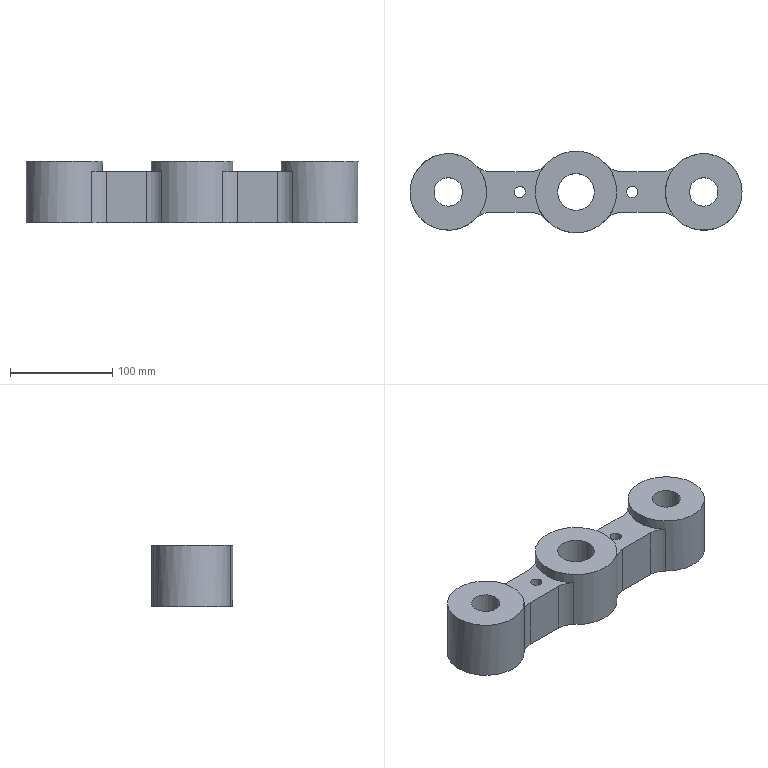Component | NX | TOP_COVER | 1 solid | 26 faces | volume 896626 mm3 | cylinder 16 | plane 10 | commonest cylinder face diameters 40 x8 75 x2 28 x2 11 x2 80 x1 36 x1